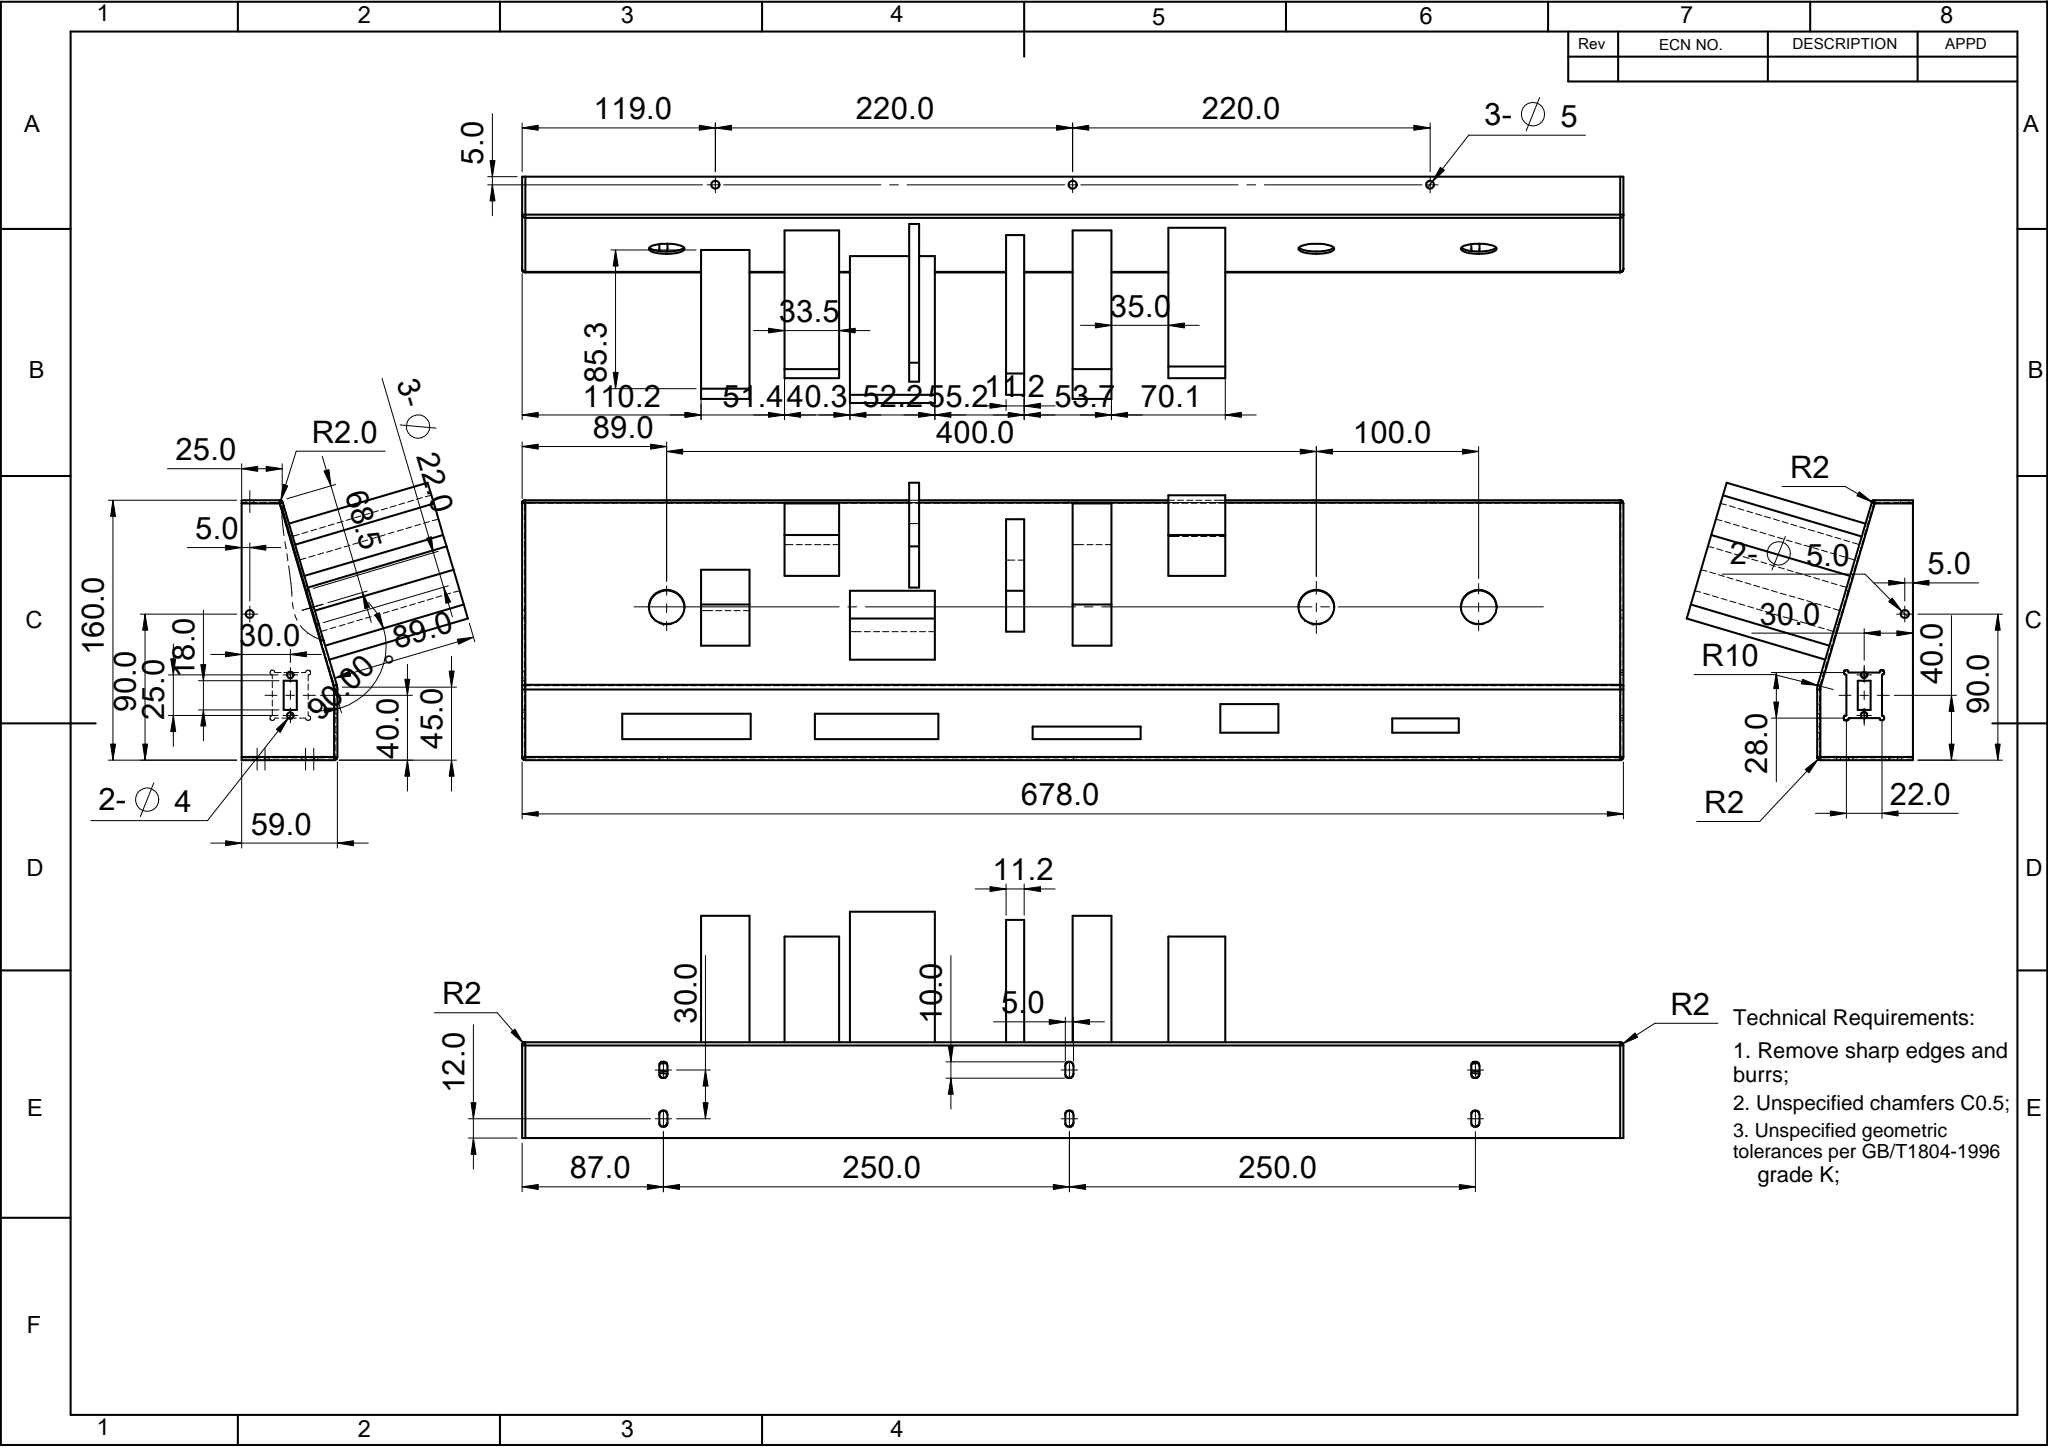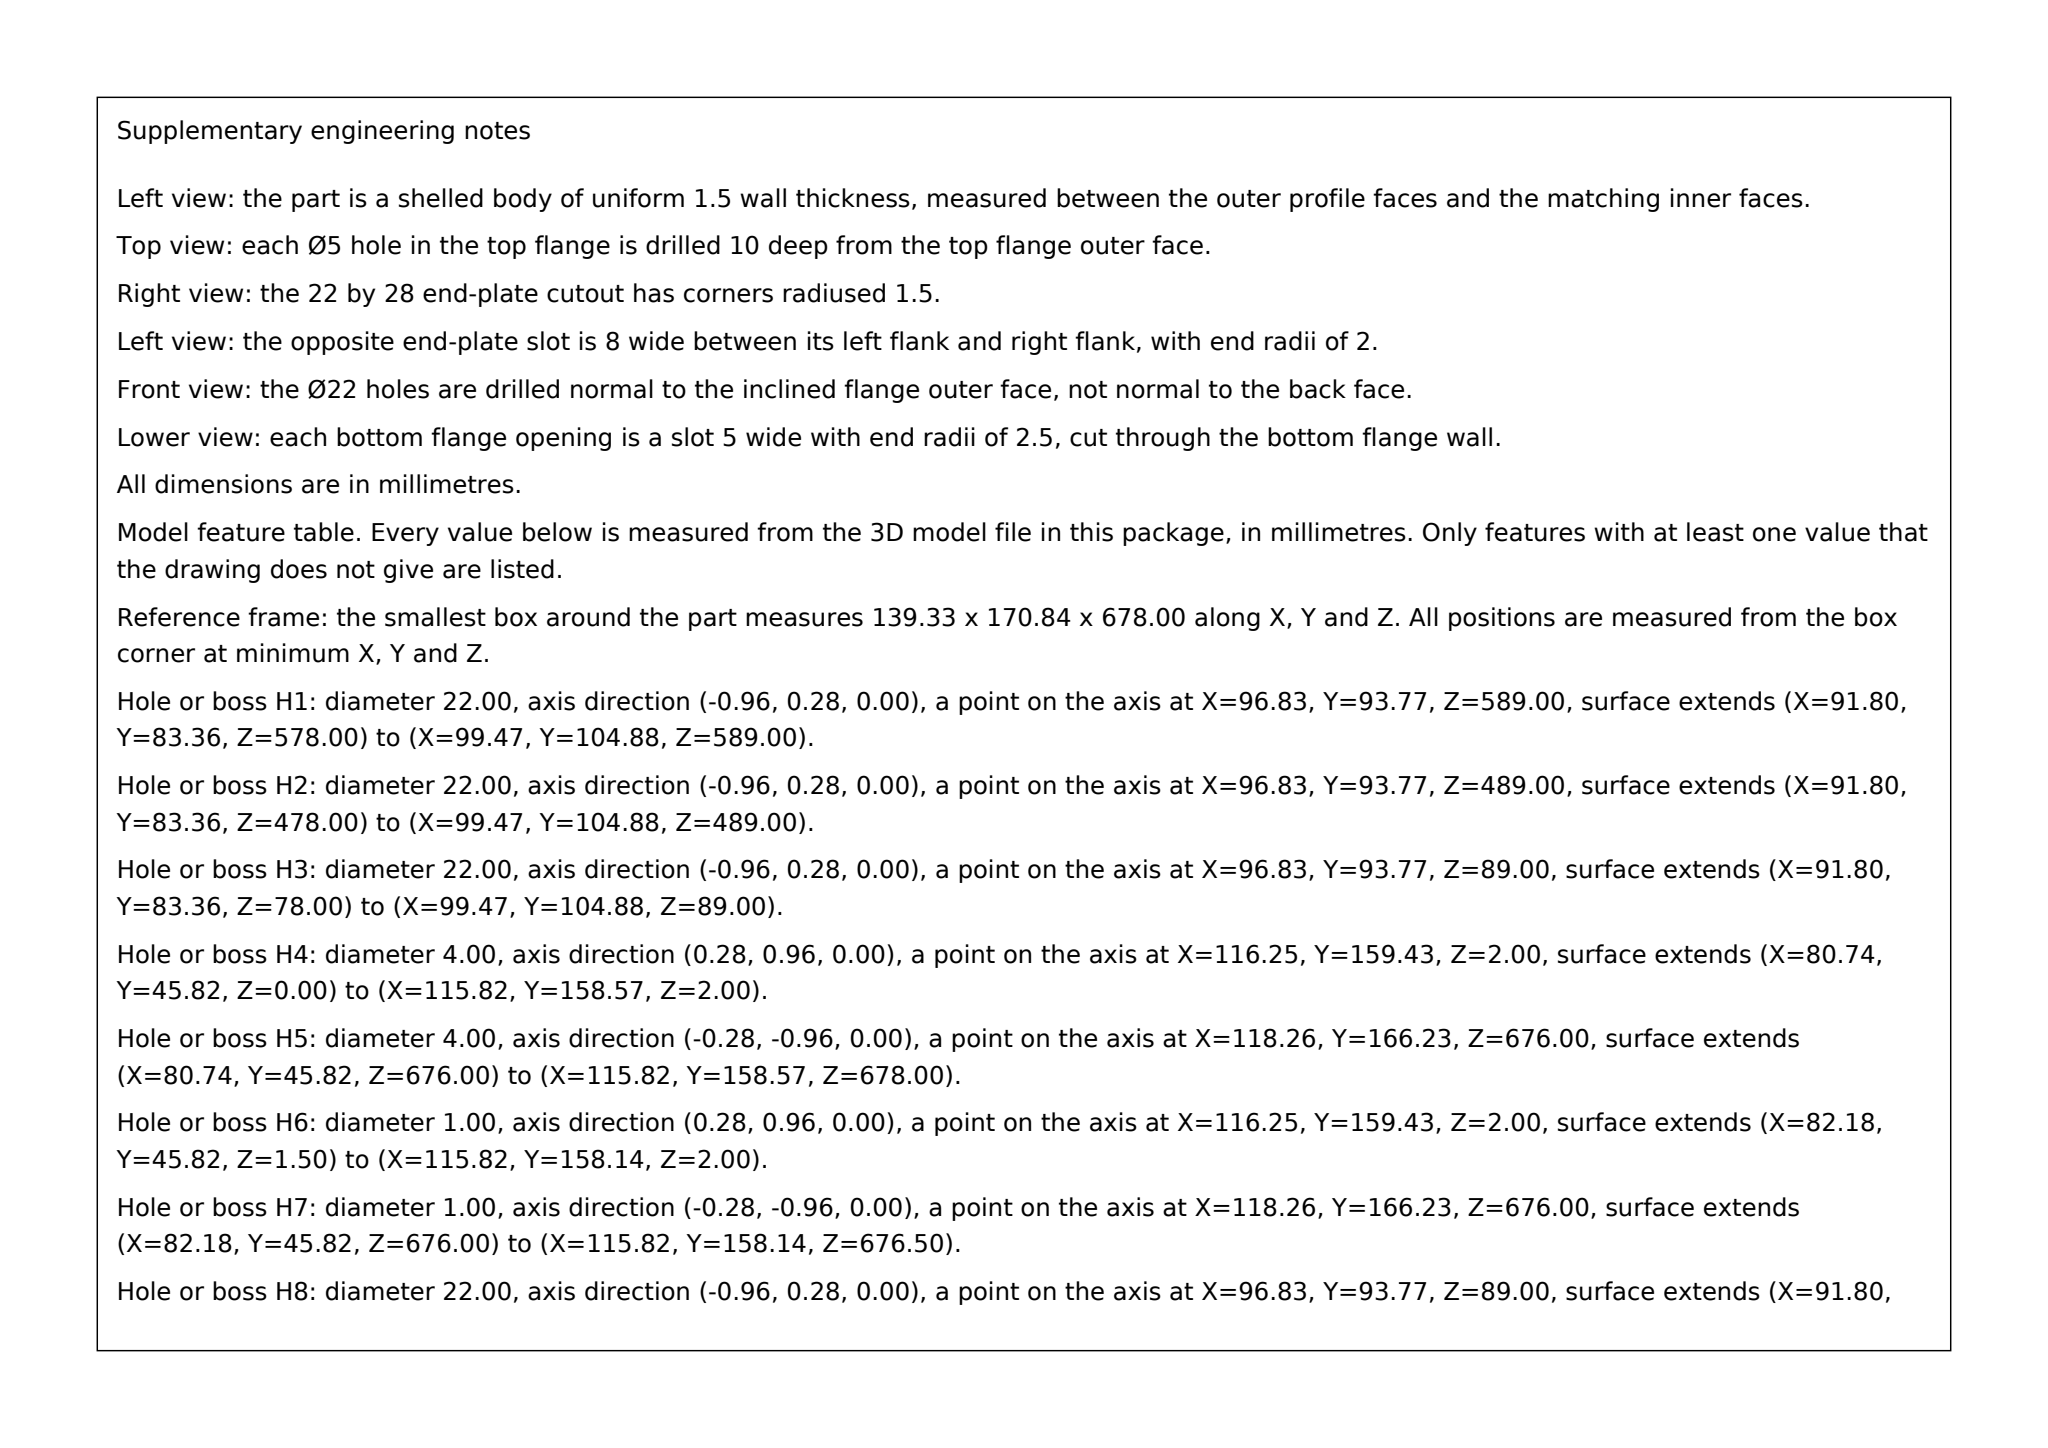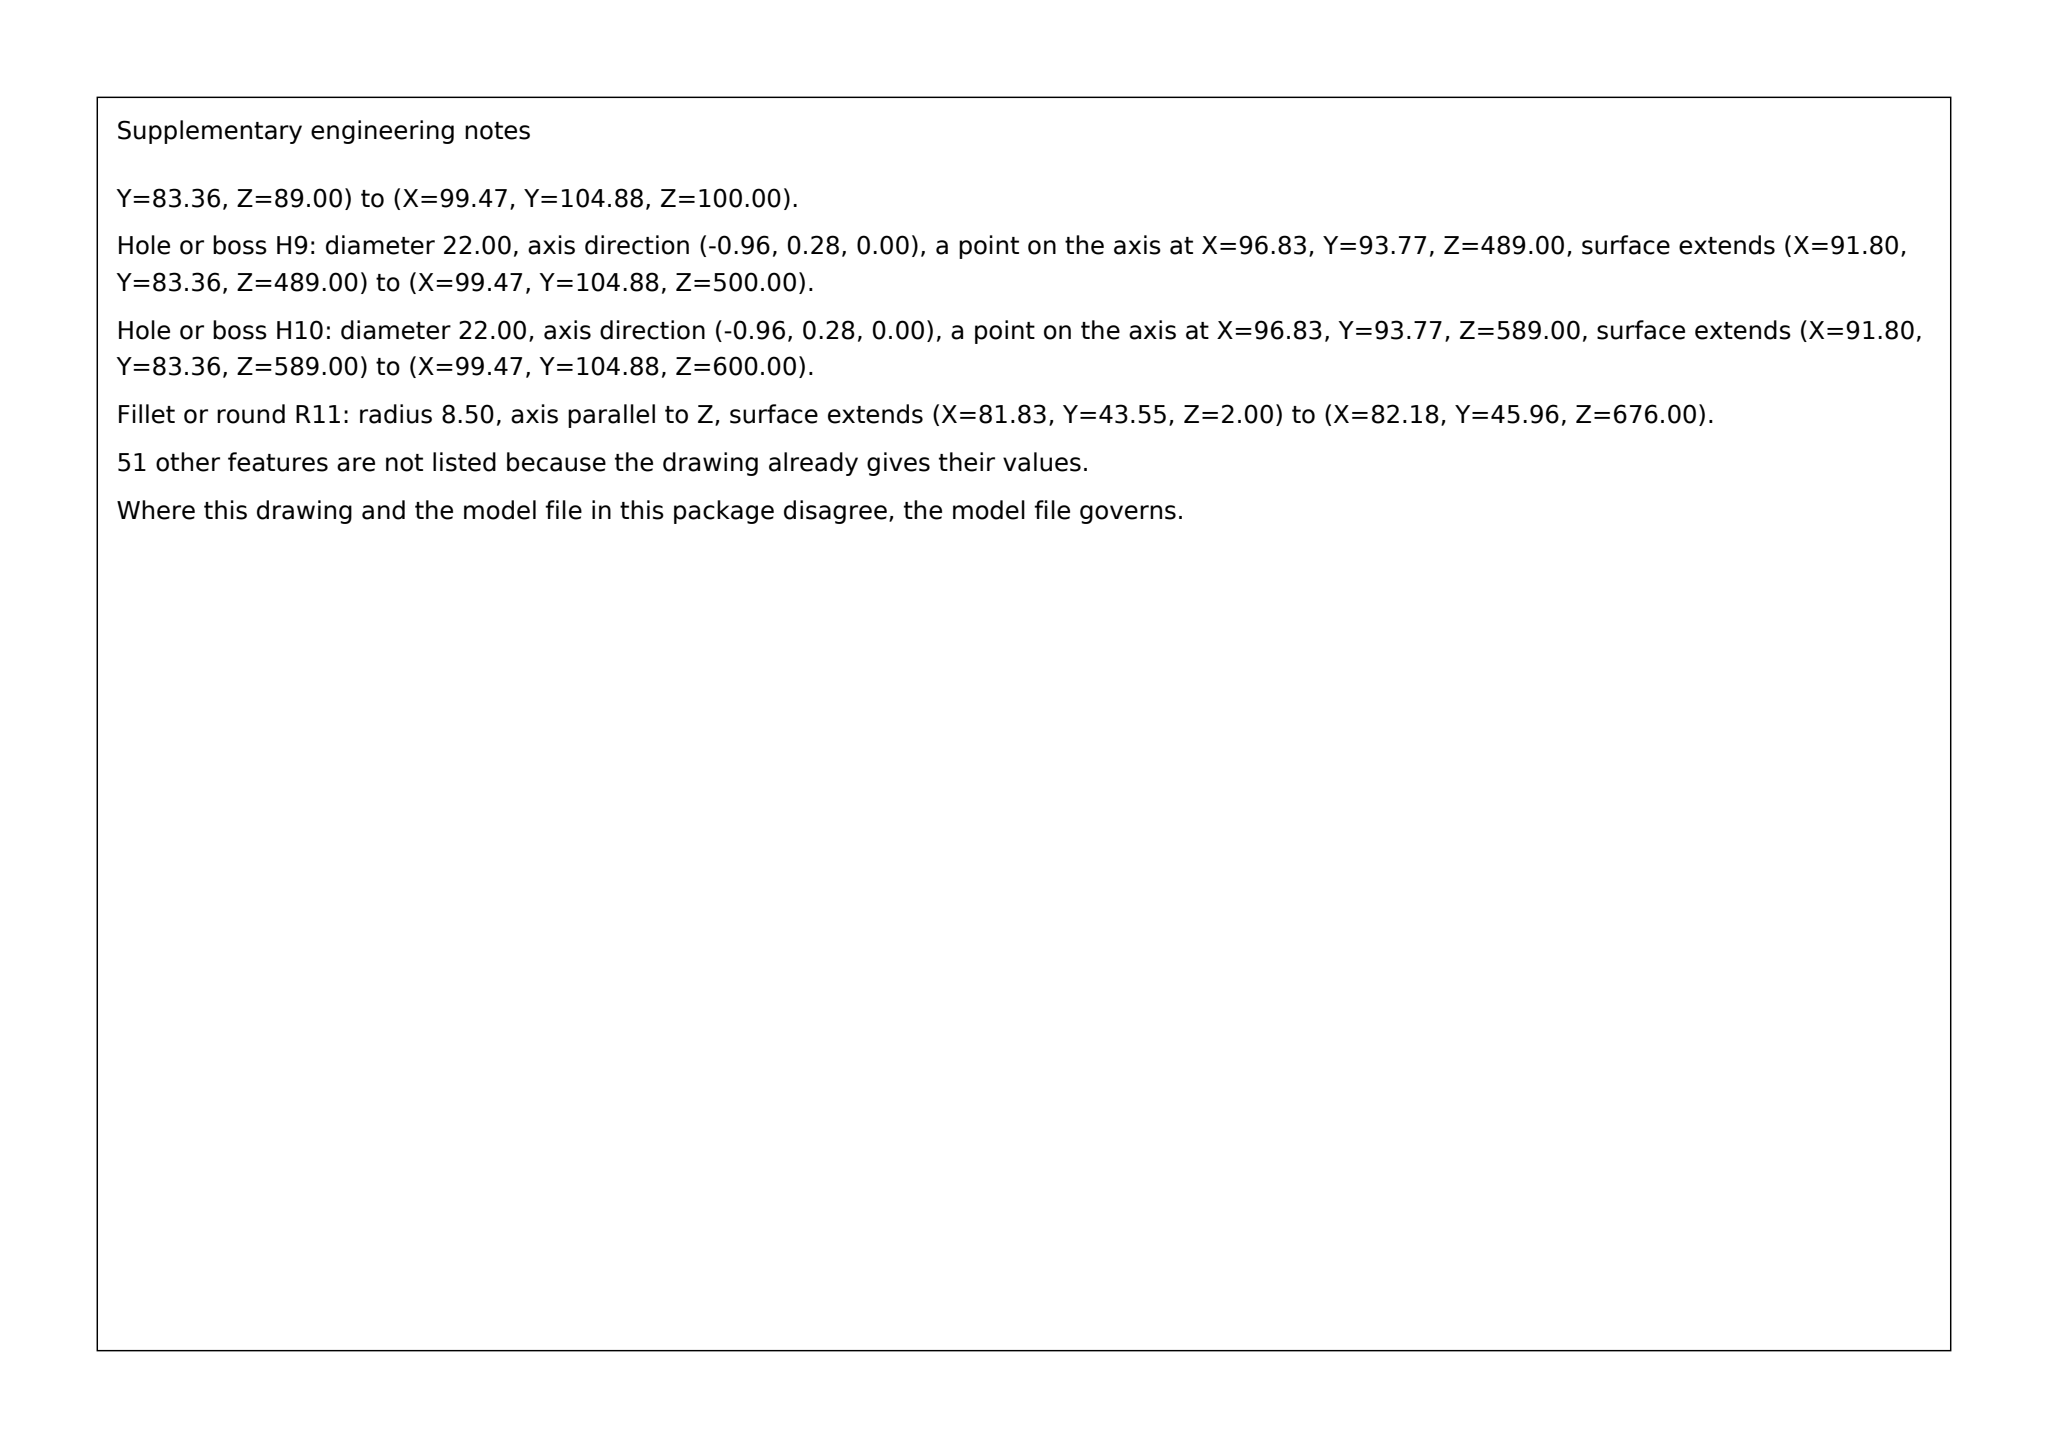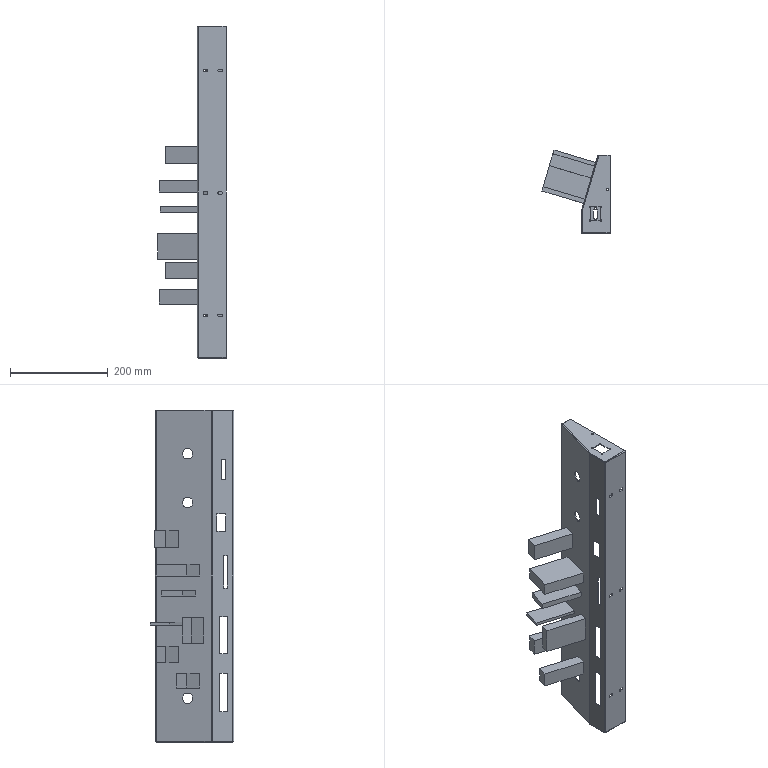Part | SolidWorks | mm | 1 solid | 166 faces | box 139.33 x 170.84 x 678 mm | volume 747545 mm3 | plane 88 | cylinder 66 | sphere 8 | torus 4 | commonest cylinder face diameters 5 x28 4 x14 1 x10 22 x6 3 x6 20 x1 17 x1
Drawing notes:
ALL DIMENSIONS IN MILLIMETRES. | from the solid: bbox_xyz given in mm [139.33, 170.838, 678.0]
MATERIAL THICKNESS 1.5 (sheet, uniform all walls). | from the solid: axis_planes y=0.0 and y=1.5 (bottom face pair); end plates z=0.0 and z=1.5
OVERALL ENVELOPE 139.3 (X) x 170.8 (Y) x 678.0 (Z). | from the solid: bbox_xyz [139.33, 170.838, 678.0]
BEND ANGLE 90 deg at base/back-flange bend, bend line at X=82.3, Y=2.0, running full length Z=2.0 to 676.0. | from the solid: convex arc dia 4.0 / concave arc dia 1.0, z axis at [82.3, 2.0], arc_deg 90
BEND ANGLE 74 deg between sloped web and top flange, bend line at X=115.8, Y=158.0, running Z=2.0 to 676.0. | from the solid: convex arc dia 4.0 / concave arc dia 1.0, z axis at [115.8, 158.0], arc_deg 74
UNSPECIFIED BEND RADII: INSIDE R0.5, OUTSIDE R2.0. Large formed bend: inside R8.5 / outside R10.0 at X=90.3, Y=43.6, 16 deg. | from the solid: concave arcs dia 1.0 / convex arcs dia 4.0 at all bend lines; concave dia 17.0 / convex dia 20.0 z axis at [90.3, 43.6]
LEFT END PLATE (Z=0 to 1.5): RECTANGULAR CUT-OUT 8.0 WIDE x 18.0 HIGH, X=105.3 to 113.3, Y=31.0 to 49.0 from bbox min corner. | from the solid: axis_planes x=105.3 and x=113.3 extent y[31.0,49.0] z[0.0,1.5]; y=31.0 and y=49.0 extent x[105.3,113.3]
RIGHT END PLATE (Z=676.5 to 678.0): RECTANGULAR CUT-OUT 22.0 WIDE x 28.0 HIGH, X=98.3 to 120.3, Y=26.0 to 54.0, 4X R1.5 CORNERS. | from the solid: axis_planes x=98.3/120.3 extent y[27.5,52.5]; y=26.0/54.0 extent x[99.8,118.8]; concave arcs dia 3.0 z axis at [98.3,26.0],[98.3,54.0],[120.3,26.0],[120.3,54.0]
1X Ø5.0 THRU IN EACH END PLATE (2 PLACES TOTAL) AT X=134.3, Y=90.0 from bbox min corner. | from the solid: hole/bore dia 5.0, z axis at [134.3, 90.0], from 0.0 to 1.5 and from 676.5 to 678.0
2X Ø4.0 THRU IN LEFT END PLATE (Z=0 to 1.5) AT X=109.3, Y=27.5 AND Y=52.5 (25.0 APART). | from the solid: hole/bore dia 4.0, z axis at [109.3, 27.5] and [109.3, 52.5], from 0.0 to 1.5
6X OBROUND SLOT 5.0 WIDE x 10.0 OVERALL (R2.5 ENDS) THRU 1.5 BOTTOM FACE; SLOT CENTRES X=97.3 AND X=127.3, AT Z=87.0, 337.0 AND 587.0. | from the solid: concave arcs dia 5.0, y axis at x=94.8/99.8 and x=124.8/129.8, at z=87.0, 337.0, 587.0, from y 0.0 to 1.5
TOP/SLOPED-FACE TAB CUT-OUT EDGES LOCATED FROM Z=0 END FACE: Z=110.2/140.0, 161.6/195.1, 201.8/254.0, 238.4/244.3, 298.0/309.2, 339.0/362.9, 397.9/432.9. | from the solid: axis_planes normal z at offsets 110.2, 140.0, 161.6, 195.1, 201.8, 238.4, 244.3, 254.0, 298.0, 309.2, 339.0, 362.9, 397.9, 432.9
BACK FLANGE (WALL X=80.3 to 81.8) RELIEFS: Z=61.7-140.7 AND Z=180.2-256.3 SPAN Y=13.0-28.6; Z=314.4-380.7 SPANS Y=13.0-20.8; Z=429.9-465.7 SPANS Y=16.9-34.6; Z=535.8-576.8 SPANS Y=16.9-25.7. | from the solid: axis_planes y=13.0, 16.9, 20.8, 25.7, 28.6 with extent x[80.3,81.8] over listed z ranges
3X Ø22.0 THRU ON SLOPED FACE, HOLE AXES AT Y=93.8, Z=89.0, 489.0 AND 589.0. | from the solid: hole/bore dia 22.0, inclined axis at [null, 93.8, 89.0 / 489.0 / 589.0], from 91.8 to 99.5
SLOPED-FACE TAB CUT-OUT AT Z=110.2 TO 140.0: ACROSS-FACE EXTENT Y=70.6 TO 117.2 FROM BBOX MIN CORNER. | from the solid: axis_plane z=110.2 and z=140.0, extent y [70.6,117.2]
SLOPED-FACE TAB CUT-OUT AT Z=161.6 TO 195.1: ACROSS-FACE EXTENT Y=113.4 TO 158.0 FROM BBOX MIN CORNER. | from the solid: axis_plane z=161.6 and z=195.1, extent y [113.4,158.0]
SLOPED-FACE TAB CUT-OUT AT Z=201.8 TO 254.0: ACROSS-FACE EXTENT Y=62.0 TO 104.4 FROM BBOX MIN CORNER. | from the solid: axis_plane z=201.8 and z=254.0, extent y [62.0,104.4]
SLOPED-FACE TAB CUT-OUT AT Z=238.4 TO 244.3: ACROSS-FACE EXTENT Y=106.3 TO 170.8 FROM BBOX MIN CORNER. | from the solid: axis_plane z=238.4 and z=244.3, extent y [106.3,170.8]
SLOPED-FACE TAB CUT-OUT AT Z=298.0 TO 309.2: ACROSS-FACE EXTENT Y=79.1 TO 148.3 FROM BBOX MIN CORNER. | from the solid: axis_plane z=298.0 and z=309.2, extent y [79.1,148.3]
SLOPED-FACE TAB CUT-OUT AT Z=339.0 TO 362.9: ACROSS-FACE EXTENT Y=70.6 TO 158.0 FROM BBOX MIN CORNER. | from the solid: axis_plane z=339.0 and z=362.9, extent y [70.6,158.0]
SLOPED-FACE TAB CUT-OUT AT Z=397.9 TO 432.9: ACROSS-FACE EXTENT Y=113.4 TO 163.0 FROM BBOX MIN CORNER. | from the solid: axis_plane z=397.9 and z=432.9, extent y [113.4,163.0]
BACK FLANGE WALL AT X=80.3 TO 81.8 (1.5 THK): HEIGHT Y=2.0 TO 43.6 (41.6 HIGH), RUNNING Z=2.0 TO 676.0 FULL LENGTH. | from the solid: axis_planes x=80.3 and x=81.8, extent y [2.0,43.6], z [2.0,676.0]
SLOPED-FACE TAB CUT-OUT WIDTHS ALONG Z (REPLACES GARBLED TOP-VIEW CHAIN): FIRST CUT-OUT EDGE AT Z=110.2 FROM Z=0 END FACE. | from the solid: axis_plane z=110.2 (first sloped-face cut face)
7X FORMED TAB ON SLOPED FACE, WIDTH ALONG Z: 29.8, 33.5, 52.2, 5.9, 11.2, 23.9, 35.0 AT TAB START Z=110.2, 161.6, 201.8, 238.4, 298.0, 339.0, 397.9 FROM Z=0 END FACE | from the solid: paired z-normal planar faces at z=110.2/140.0, 161.6/195.1, 201.8/254.0, 238.4/244.3, 298.0/309.2, 339.0/362.9, 397.9/432.9
TAB AT Z=110.2-140.0: PROFILE EXTENT X=2.5 TO 94.2, Y=70.6 TO 117.2 FROM BBOX MIN CORNER | from the solid: axis_planes z=110.2 and z=140.0, extent x[2.5,94.2] y[70.6,117.2]
TAB AT Z=161.6-195.1: PROFILE EXTENT X=15.2 TO 106.3, Y=113.4 TO 158.0 FROM BBOX MIN CORNER | from the solid: axis_planes z=161.6 and z=195.1, extent x[15.2,106.3] y[113.4,158.0]
TAB AT Z=201.8-254.0: PROFILE EXTENT X=0.0 TO 90.4, Y=62.0 TO 104.4 FROM BBOX MIN CORNER | from the solid: axis_planes z=201.8 and z=254.0, extent x[0.0,90.4] y[62.0,104.4]
TAB AT Z=238.4-244.3: PROFILE EXTENT X=13.1 TO 110.1, Y=106.3 TO 170.8 FROM BBOX MIN CORNER | from the solid: axis_planes z=238.4 and z=244.3, extent x[13.1,110.1] y[106.3,170.8]
TAB AT Z=298.0-309.2: PROFILE EXTENT X=5.1 TO 103.4, Y=79.1 TO 148.3 FROM BBOX MIN CORNER | from the solid: axis_planes z=298.0 and z=309.2, extent x[5.1,103.4] y[79.1,148.3]
TAB AT Z=339.0-362.9: PROFILE EXTENT X=2.5 TO 106.3, Y=70.6 TO 158.0 FROM BBOX MIN CORNER | from the solid: axis_planes z=339.0 and z=362.9, extent x[2.5,106.3] y[70.6,158.0]
TAB AT Z=397.9-432.9: PROFILE EXTENT X=15.2 TO 107.7, Y=113.4 TO 163.0 FROM BBOX MIN CORNER | from the solid: axis_planes z=397.9 and z=432.9, extent x[15.2,107.7] y[113.4,163.0]
LEFT END PLATE CUT-OUT 8.0 WIDE (X=105.3 TO 113.3) x 18.0 HIGH (Y=31.0 TO 49.0): SHARP CORNERS, NO CORNER RADII | from the solid: left end plate cut-out bounded only by planes x=105.3, x=113.3, y=31.0, y=49.0 with no corner arc cylinders (cf. right end plate R1.5 arcs dia 3.0 at z=676.5-678.0)